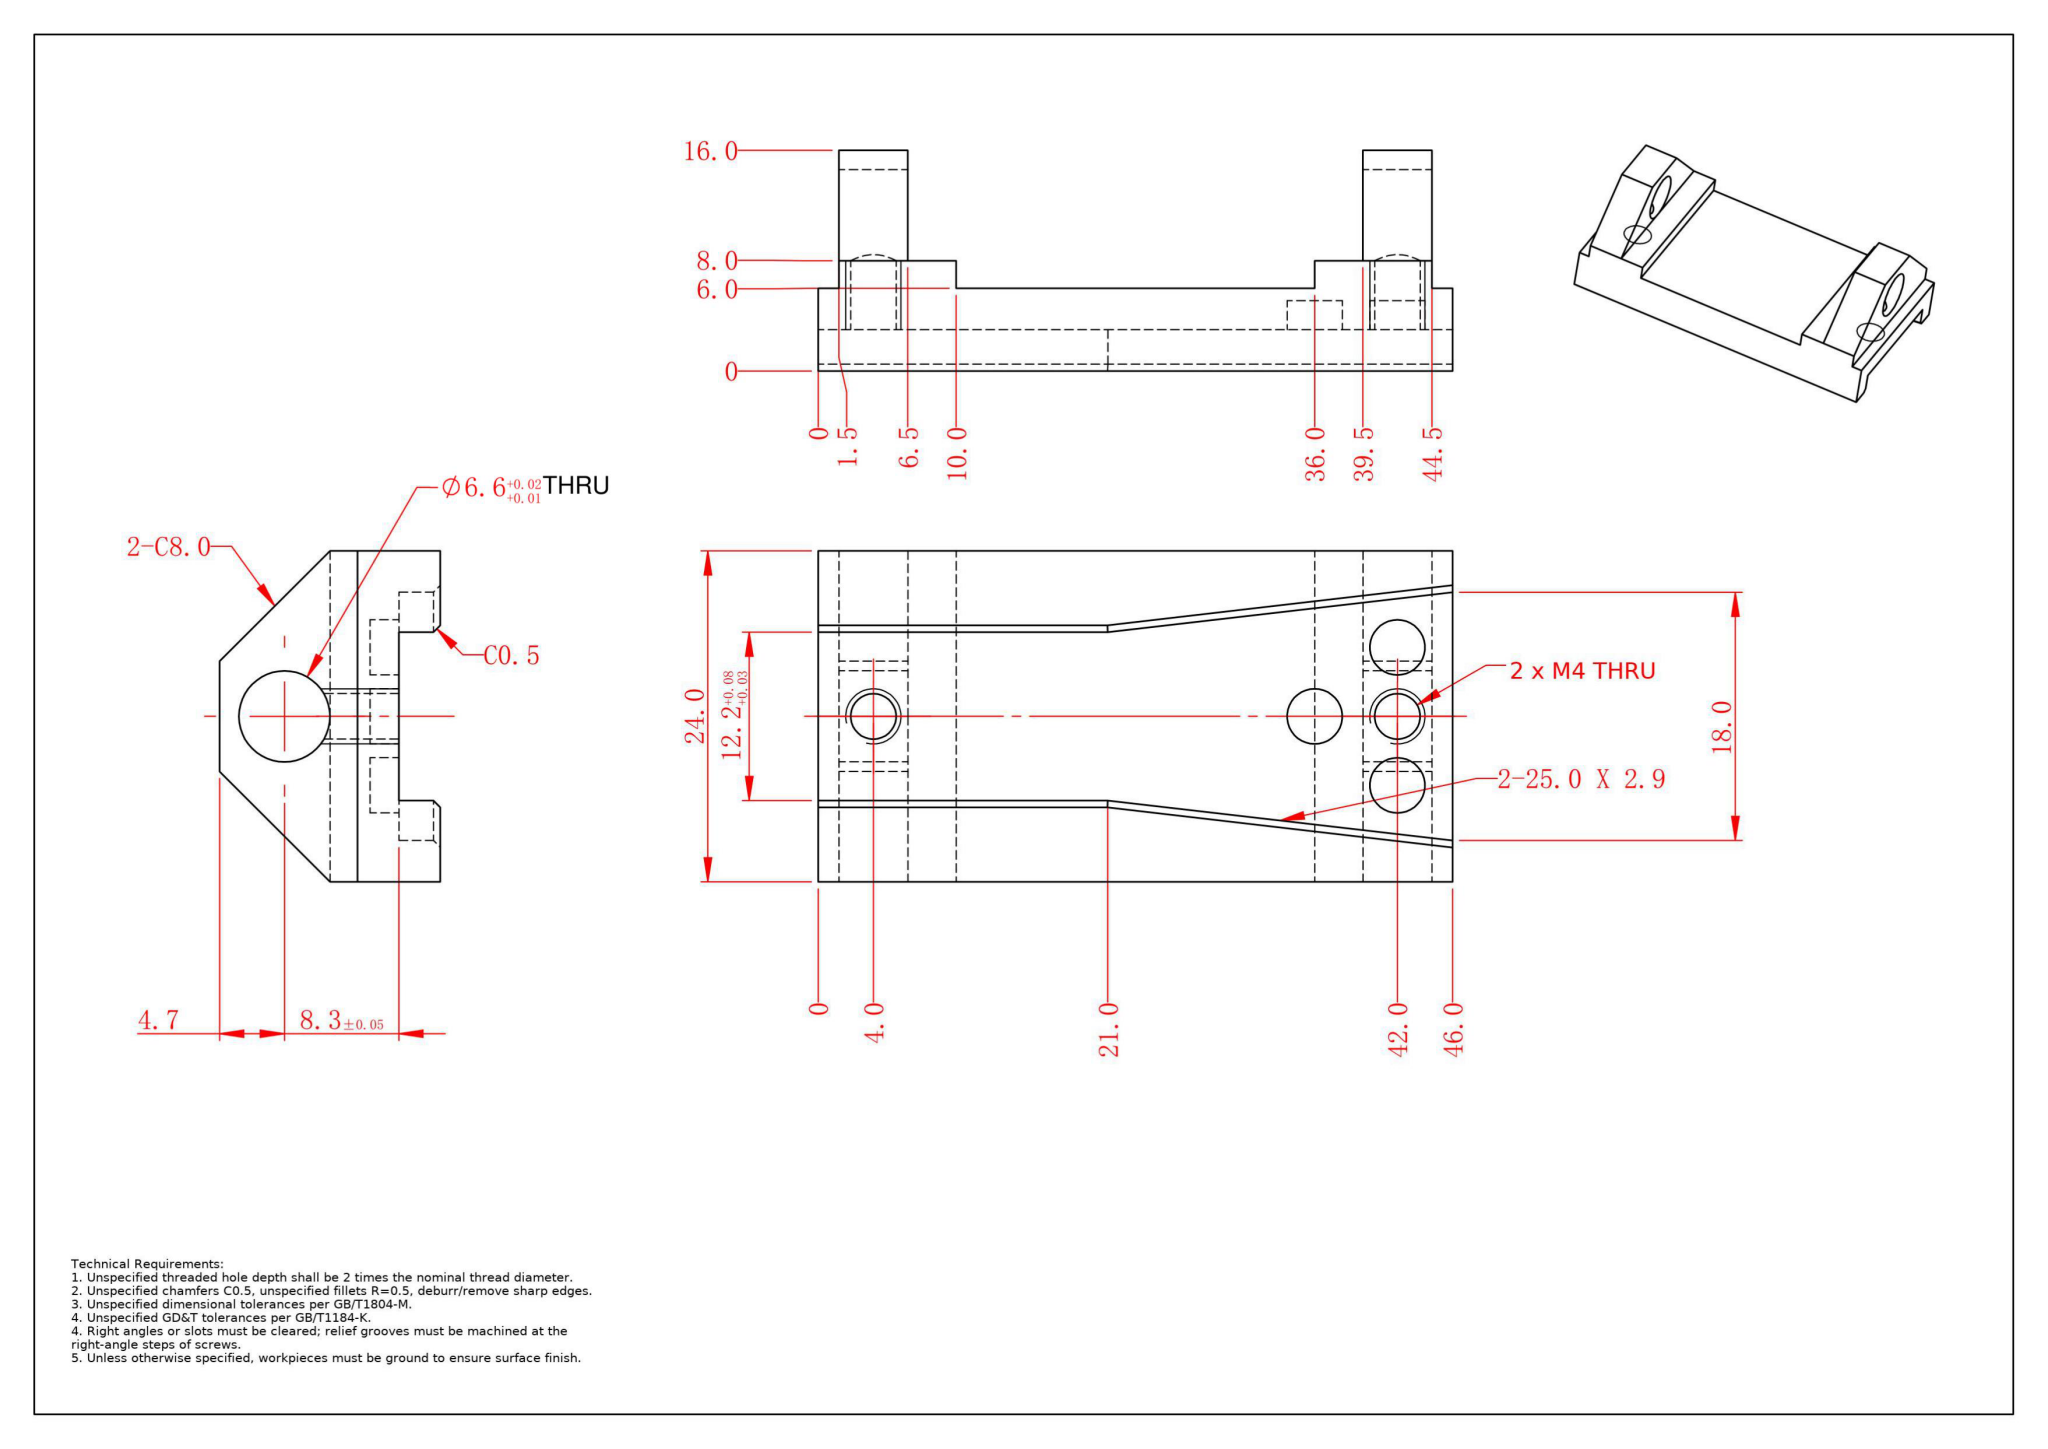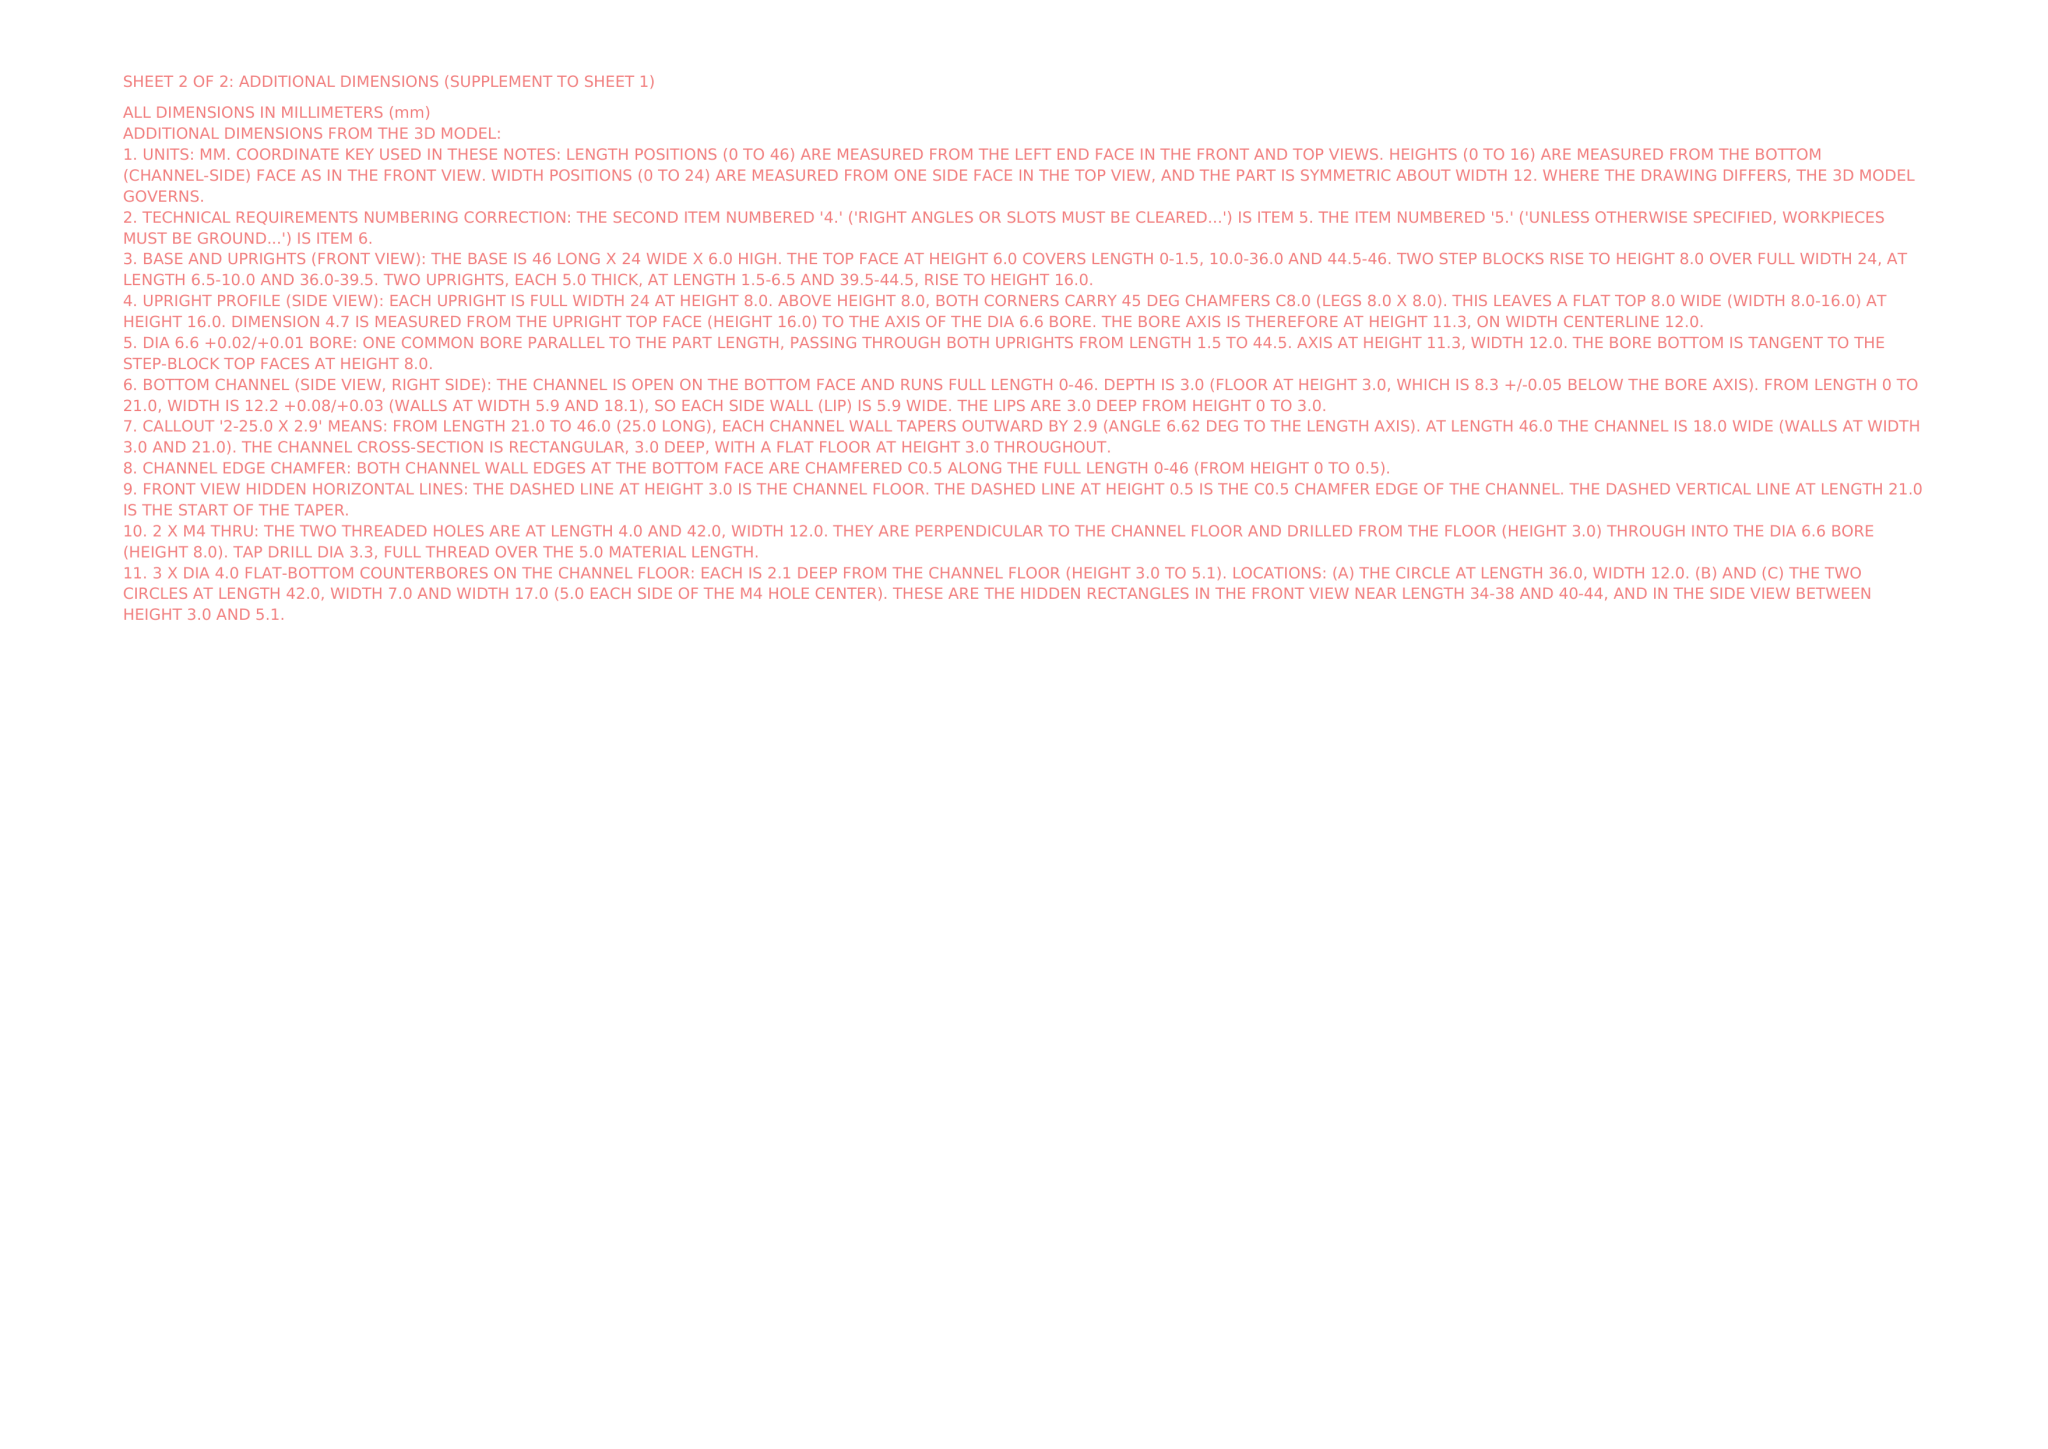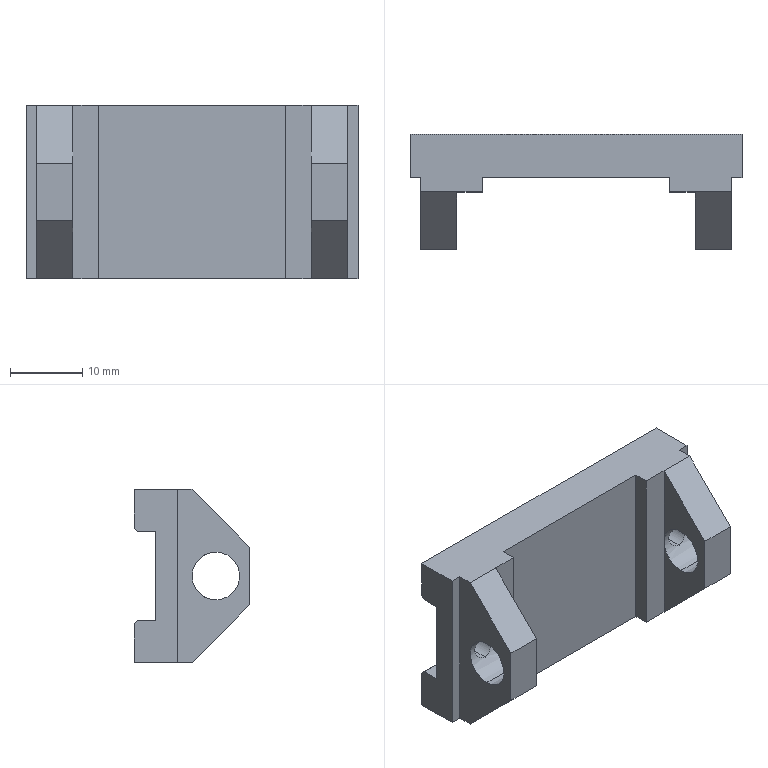Part | NX | mm | Twin-Pedestal Bore Housing Bracket | 1 solid | 49 faces | box 46 x 16 x 24 mm | volume 6299 mm3 | plane 35 | cylinder 14 | commonest cylinder face diameters 4 x6 3.3 x4 6.6 x4